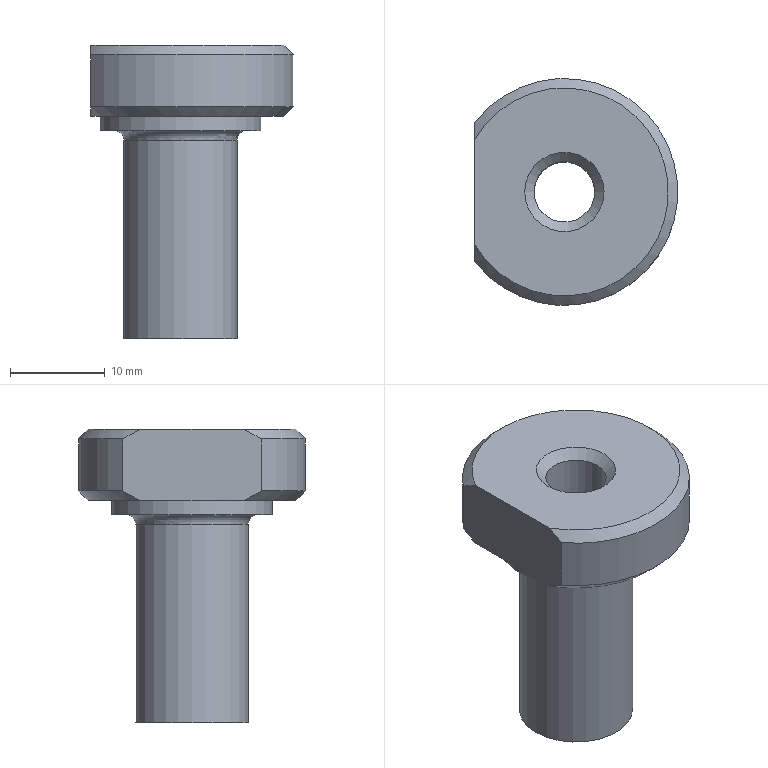Component | NX | GUIDE_BUSH_1 | 1 solid | 14 faces | box 21.5 x 24 x 31 mm | volume 4964 mm3 | plane 5 | cylinder 4 | cone 4 | torus 1 | commonest cylinder face diameters 12 x1 17 x1 24 x1 6.4 x1
STEP:
#1=CARTESIAN_POINT('',(0.,0.,0.));
#2=DIRECTION('',(0.,0.,1.));
#3=DIRECTION('',(1.,0.,0.));
#4=AXIS2_PLACEMENT_3D('',#1,#2,#3);
#5=CARTESIAN_POINT('',(-4.2,-1.,124.5));
#6=VERTEX_POINT('',#5);
#7=CARTESIAN_POINT('',(0.,-1.,124.5));
#8=DIRECTION('',(0.,0.,1.));
#9=DIRECTION('',(-1.,0.,0.));
#10=AXIS2_PLACEMENT_3D('',#7,#8,#9);
#11=CIRCLE('',#10,4.2);
#12=CARTESIAN_POINT('',(6.,-1.,124.5));
#13=DIRECTION('',(0.,0.,-1.));
#14=DIRECTION('',(-1.,0.,0.));
#15=AXIS2_PLACEMENT_3D('',#12,#13,#14);
#16=PLANE('',#15);
#17=CARTESIAN_POINT('',(10.2,0.));
#18=CARTESIAN_POINT('',(10.2,-7.275));
#19=CARTESIAN_POINT('',(3.9,-3.637));
#20=CARTESIAN_POINT('',(-2.4,-0.));
#21=CARTESIAN_POINT('',(3.9,3.637));
#22=CARTESIAN_POINT('',(10.2,7.275));
#23=CARTESIAN_POINT('',(10.2,0.));
#24=(BOUNDED_CURVE()B_SPLINE_CURVE(2,(#17,#18,#19,#20,#21,#22,#23),.UNSPECIFIED.,.T.,.F.)B_SPLINE_CURVE_WITH_KNOTS((1,2,2,2,2,1),(-2.094,0.,2.094,4.189,6.283,8.378),.UNSPECIFIED.)CURVE()GEOMETRIC_REPRESENTATION_ITEM()RATIONAL_B_SPLINE_CURVE((1.,0.5,1.,0.5,1.,0.5,1.))REPRESENTATION_ITEM(''));
#25=(GEOMETRIC_REPRESENTATION_CONTEXT(2)PARAMETRIC_REPRESENTATION_CONTEXT()REPRESENTATION_CONTEXT('',''));
#26=DEFINITIONAL_REPRESENTATION('',(#24),#25);
#27=PCURVE('',#16,#26);
#28=CARTESIAN_POINT('',(0.,-1.,124.5));
#29=DIRECTION('',(0.,0.,-1.));
#30=DIRECTION('',(-1.,0.,0.));
#31=AXIS2_PLACEMENT_3D('',#28,#29,#30);
#32=CONICAL_SURFACE('',#31,4.2,0.7854);
#33=CARTESIAN_POINT('',(6.283,0.));
#34=DIRECTION('',(-1.,0.));
#35=VECTOR('',#34,1.);
#36=LINE('',#33,#35);
#37=(GEOMETRIC_REPRESENTATION_CONTEXT(2)PARAMETRIC_REPRESENTATION_CONTEXT()REPRESENTATION_CONTEXT('',''));
#38=DEFINITIONAL_REPRESENTATION('',(#36),#37);
#39=PCURVE('',#32,#38);
#40=SURFACE_CURVE('',#11,(#27,#39),.PCURVE_S1.);
#41=EDGE_CURVE('',#6,#6,#40,.T.);
#42=ORIENTED_EDGE('',*,*,#41,.T.);
#43=EDGE_LOOP('',(#42));
#44=FACE_BOUND('',#43,.T.);
#45=CARTESIAN_POINT('',(6.,-1.,124.5));
#46=VERTEX_POINT('',#45);
#47=CARTESIAN_POINT('',(0.,-1.,124.5));
#48=DIRECTION('',(0.,0.,1.));
#49=DIRECTION('',(1.,0.,0.));
#50=AXIS2_PLACEMENT_3D('',#47,#48,#49);
#51=CIRCLE('',#50,6.);
#52=CARTESIAN_POINT('',(0.,0.));
#53=CARTESIAN_POINT('',(0.,10.392));
#54=CARTESIAN_POINT('',(9.,5.196));
#55=CARTESIAN_POINT('',(18.,0.));
#56=CARTESIAN_POINT('',(9.,-5.196));
#57=CARTESIAN_POINT('',(0.,-10.392));
#58=CARTESIAN_POINT('',(0.,0.));
#59=(BOUNDED_CURVE()B_SPLINE_CURVE(2,(#52,#53,#54,#55,#56,#57,#58),.UNSPECIFIED.,.T.,.F.)B_SPLINE_CURVE_WITH_KNOTS((1,2,2,2,2,1),(-2.094,0.,2.094,4.189,6.283,8.378),.UNSPECIFIED.)CURVE()GEOMETRIC_REPRESENTATION_ITEM()RATIONAL_B_SPLINE_CURVE((1.,0.5,1.,0.5,1.,0.5,1.))REPRESENTATION_ITEM(''));
#60=(GEOMETRIC_REPRESENTATION_CONTEXT(2)PARAMETRIC_REPRESENTATION_CONTEXT()REPRESENTATION_CONTEXT('',''));
#61=DEFINITIONAL_REPRESENTATION('',(#59),#60);
#62=PCURVE('',#16,#61);
#63=CARTESIAN_POINT('',(0.,-1.,124.5));
#64=DIRECTION('',(0.,0.,1.));
#65=DIRECTION('',(1.,0.,0.));
#66=AXIS2_PLACEMENT_3D('',#63,#64,#65);
#67=CYLINDRICAL_SURFACE('',#66,6.);
#68=CARTESIAN_POINT('',(0.,0.));
#69=DIRECTION('',(1.,0.));
#70=VECTOR('',#69,1.);
#71=LINE('',#68,#70);
#72=(GEOMETRIC_REPRESENTATION_CONTEXT(2)PARAMETRIC_REPRESENTATION_CONTEXT()REPRESENTATION_CONTEXT('',''));
#73=DEFINITIONAL_REPRESENTATION('',(#71),#72);
#74=PCURVE('',#67,#73);
#75=SURFACE_CURVE('',#51,(#62,#74),.PCURVE_S1.);
#76=EDGE_CURVE('',#46,#46,#75,.T.);
#77=ORIENTED_EDGE('',*,*,#76,.F.);
#78=EDGE_LOOP('',(#77));
#79=FACE_BOUND('',#78,.T.);
#80=ADVANCED_FACE('',(#44,#79),#16,.T.);
#81=CARTESIAN_POINT('',(-6.,-1.,145.5));
#82=VERTEX_POINT('',#81);
#83=CARTESIAN_POINT('',(6.,-1.,145.5));
#84=VERTEX_POINT('',#83);
#85=CARTESIAN_POINT('',(0.,-1.,145.5));
#86=DIRECTION('',(0.,0.,-1.));
#87=DIRECTION('',(-1.,0.,0.));
#88=AXIS2_PLACEMENT_3D('',#85,#86,#87);
#89=CIRCLE('',#88,6.);
#90=CARTESIAN_POINT('',(3.142,21.));
#91=DIRECTION('',(-1.,0.));
#92=VECTOR('',#91,1.);
#93=LINE('',#90,#92);
#94=(GEOMETRIC_REPRESENTATION_CONTEXT(2)PARAMETRIC_REPRESENTATION_CONTEXT()REPRESENTATION_CONTEXT('',''));
#95=DEFINITIONAL_REPRESENTATION('',(#93),#94);
#96=PCURVE('',#67,#95);
#97=CARTESIAN_POINT('',(0.,-1.,145.5));
#98=DIRECTION('',(0.,0.,-1.));
#99=DIRECTION('',(-1.,0.,0.));
#100=AXIS2_PLACEMENT_3D('',#97,#98,#99);
#101=TOROIDAL_SURFACE('',#100,7.,1.);
#102=CARTESIAN_POINT('',(0.,3.142));
#103=DIRECTION('',(1.,0.));
#104=VECTOR('',#103,1.);
#105=LINE('',#102,#104);
#106=(GEOMETRIC_REPRESENTATION_CONTEXT(2)PARAMETRIC_REPRESENTATION_CONTEXT()REPRESENTATION_CONTEXT('',''));
#107=DEFINITIONAL_REPRESENTATION('',(#105),#106);
#108=PCURVE('',#101,#107);
#109=SURFACE_CURVE('',#89,(#96,#108),.PCURVE_S1.);
#110=EDGE_CURVE('',#82,#84,#109,.T.);
#111=ORIENTED_EDGE('',*,*,#110,.T.);
#112=CARTESIAN_POINT('',(6.,-1.,124.5));
#113=CARTESIAN_POINT('',(6.,-1.,145.5));
#114=B_SPLINE_CURVE_WITH_KNOTS('',1,(#112,#113),.UNSPECIFIED.,.F.,.F.,(2,2),(0.,21.),.PIECEWISE_BEZIER_KNOTS.);
#115=CARTESIAN_POINT('',(0.,0.));
#116=DIRECTION('',(0.,1.));
#117=VECTOR('',#116,1.);
#118=LINE('',#115,#117);
#119=(GEOMETRIC_REPRESENTATION_CONTEXT(2)PARAMETRIC_REPRESENTATION_CONTEXT()REPRESENTATION_CONTEXT('',''));
#120=DEFINITIONAL_REPRESENTATION('',(#118),#119);
#121=PCURVE('',#67,#120);
#122=CARTESIAN_POINT('',(6.283,0.));
#123=DIRECTION('',(0.,1.));
#124=VECTOR('',#123,1.);
#125=LINE('',#122,#124);
#126=(GEOMETRIC_REPRESENTATION_CONTEXT(2)PARAMETRIC_REPRESENTATION_CONTEXT()REPRESENTATION_CONTEXT('',''));
#127=DEFINITIONAL_REPRESENTATION('',(#125),#126);
#128=PCURVE('',#67,#127);
#129=SEAM_CURVE('',#114,(#121,#128),.PCURVE_S1.);
#130=EDGE_CURVE('',#46,#84,#129,.T.);
#131=ORIENTED_EDGE('',*,*,#130,.F.);
#132=ORIENTED_EDGE('',*,*,#76,.T.);
#133=ORIENTED_EDGE('',*,*,#130,.T.);
#134=CARTESIAN_POINT('',(0.,-1.,145.5));
#135=DIRECTION('',(0.,0.,-1.));
#136=DIRECTION('',(-1.,0.,0.));
#137=AXIS2_PLACEMENT_3D('',#134,#135,#136);
#138=CIRCLE('',#137,6.);
#139=CARTESIAN_POINT('',(9.425,21.));
#140=DIRECTION('',(-1.,0.));
#141=VECTOR('',#140,1.);
#142=LINE('',#139,#141);
#143=(GEOMETRIC_REPRESENTATION_CONTEXT(2)PARAMETRIC_REPRESENTATION_CONTEXT()REPRESENTATION_CONTEXT('',''));
#144=DEFINITIONAL_REPRESENTATION('',(#142),#143);
#145=PCURVE('',#67,#144);
#146=CARTESIAN_POINT('',(0.,3.142));
#147=DIRECTION('',(1.,0.));
#148=VECTOR('',#147,1.);
#149=LINE('',#146,#148);
#150=(GEOMETRIC_REPRESENTATION_CONTEXT(2)PARAMETRIC_REPRESENTATION_CONTEXT()REPRESENTATION_CONTEXT('',''));
#151=DEFINITIONAL_REPRESENTATION('',(#149),#150);
#152=PCURVE('',#101,#151);
#153=SURFACE_CURVE('',#138,(#145,#152),.PCURVE_S1.);
#154=EDGE_CURVE('',#84,#82,#153,.T.);
#155=ORIENTED_EDGE('',*,*,#154,.T.);
#156=EDGE_LOOP('',(#111,#131,#132,#133,#155));
#157=FACE_BOUND('',#156,.T.);
#158=ADVANCED_FACE('',(#157),#67,.T.);
#159=CARTESIAN_POINT('',(-7.,-1.,146.5));
#160=VERTEX_POINT('',#159);
#161=CARTESIAN_POINT('',(0.,-1.,146.5));
#162=DIRECTION('',(0.,0.,1.));
#163=DIRECTION('',(-1.,0.,0.));
#164=AXIS2_PLACEMENT_3D('',#161,#162,#163);
#165=CIRCLE('',#164,7.);
#166=CARTESIAN_POINT('',(8.5,-1.,146.5));
#167=DIRECTION('',(0.,0.,-1.));
#168=DIRECTION('',(-1.,0.,0.));
#169=AXIS2_PLACEMENT_3D('',#166,#167,#168);
#170=PLANE('',#169);
#171=CARTESIAN_POINT('',(15.5,0.));
#172=CARTESIAN_POINT('',(15.5,-12.124));
#173=CARTESIAN_POINT('',(5.,-6.062));
#174=CARTESIAN_POINT('',(-5.5,-0.));
#175=CARTESIAN_POINT('',(5.,6.062));
#176=CARTESIAN_POINT('',(15.5,12.124));
#177=CARTESIAN_POINT('',(15.5,0.));
#178=(BOUNDED_CURVE()B_SPLINE_CURVE(2,(#171,#172,#173,#174,#175,#176,#177),.UNSPECIFIED.,.T.,.F.)B_SPLINE_CURVE_WITH_KNOTS((1,2,2,2,2,1),(-2.094,0.,2.094,4.189,6.283,8.378),.UNSPECIFIED.)CURVE()GEOMETRIC_REPRESENTATION_ITEM()RATIONAL_B_SPLINE_CURVE((1.,0.5,1.,0.5,1.,0.5,1.))REPRESENTATION_ITEM(''));
#179=(GEOMETRIC_REPRESENTATION_CONTEXT(2)PARAMETRIC_REPRESENTATION_CONTEXT()REPRESENTATION_CONTEXT('',''));
#180=DEFINITIONAL_REPRESENTATION('',(#178),#179);
#181=PCURVE('',#170,#180);
#182=CARTESIAN_POINT('',(6.283,4.712));
#183=DIRECTION('',(-1.,0.));
#184=VECTOR('',#183,1.);
#185=LINE('',#182,#184);
#186=(GEOMETRIC_REPRESENTATION_CONTEXT(2)PARAMETRIC_REPRESENTATION_CONTEXT()REPRESENTATION_CONTEXT('',''));
#187=DEFINITIONAL_REPRESENTATION('',(#185),#186);
#188=PCURVE('',#101,#187);
#189=SURFACE_CURVE('',#165,(#181,#188),.PCURVE_S1.);
#190=EDGE_CURVE('',#160,#160,#189,.T.);
#191=ORIENTED_EDGE('',*,*,#190,.T.);
#192=EDGE_LOOP('',(#191));
#193=FACE_BOUND('',#192,.T.);
#194=CARTESIAN_POINT('',(8.5,-1.,146.5));
#195=VERTEX_POINT('',#194);
#196=CARTESIAN_POINT('',(0.,-1.,146.5));
#197=DIRECTION('',(0.,0.,1.));
#198=DIRECTION('',(1.,0.,0.));
#199=AXIS2_PLACEMENT_3D('',#196,#197,#198);
#200=CIRCLE('',#199,8.5);
#201=CARTESIAN_POINT('',(0.,0.));
#202=CARTESIAN_POINT('',(0.,14.722));
#203=CARTESIAN_POINT('',(12.75,7.361));
#204=CARTESIAN_POINT('',(25.5,0.));
#205=CARTESIAN_POINT('',(12.75,-7.361));
#206=CARTESIAN_POINT('',(0.,-14.722));
#207=CARTESIAN_POINT('',(0.,0.));
#208=(BOUNDED_CURVE()B_SPLINE_CURVE(2,(#201,#202,#203,#204,#205,#206,#207),.UNSPECIFIED.,.T.,.F.)B_SPLINE_CURVE_WITH_KNOTS((1,2,2,2,2,1),(-2.094,0.,2.094,4.189,6.283,8.378),.UNSPECIFIED.)CURVE()GEOMETRIC_REPRESENTATION_ITEM()RATIONAL_B_SPLINE_CURVE((1.,0.5,1.,0.5,1.,0.5,1.))REPRESENTATION_ITEM(''));
#209=(GEOMETRIC_REPRESENTATION_CONTEXT(2)PARAMETRIC_REPRESENTATION_CONTEXT()REPRESENTATION_CONTEXT('',''));
#210=DEFINITIONAL_REPRESENTATION('',(#208),#209);
#211=PCURVE('',#170,#210);
#212=CARTESIAN_POINT('',(0.,-1.,124.5));
#213=DIRECTION('',(0.,0.,1.));
#214=DIRECTION('',(1.,0.,0.));
#215=AXIS2_PLACEMENT_3D('',#212,#213,#214);
#216=CYLINDRICAL_SURFACE('',#215,8.5);
#217=CARTESIAN_POINT('',(0.,22.));
#218=DIRECTION('',(1.,0.));
#219=VECTOR('',#218,1.);
#220=LINE('',#217,#219);
#221=(GEOMETRIC_REPRESENTATION_CONTEXT(2)PARAMETRIC_REPRESENTATION_CONTEXT()REPRESENTATION_CONTEXT('',''));
#222=DEFINITIONAL_REPRESENTATION('',(#220),#221);
#223=PCURVE('',#216,#222);
#224=SURFACE_CURVE('',#200,(#211,#223),.PCURVE_S1.);
#225=EDGE_CURVE('',#195,#195,#224,.T.);
#226=ORIENTED_EDGE('',*,*,#225,.F.);
#227=EDGE_LOOP('',(#226));
#228=FACE_BOUND('',#227,.T.);
#229=ADVANCED_FACE('',(#193,#228),#170,.T.);
#230=ORIENTED_EDGE('',*,*,#225,.T.);
#231=CARTESIAN_POINT('',(8.5,-1.,148.));
#232=VERTEX_POINT('',#231);
#233=CARTESIAN_POINT('',(8.5,-1.,146.5));
#234=CARTESIAN_POINT('',(8.5,-1.,148.));
#235=B_SPLINE_CURVE_WITH_KNOTS('',1,(#233,#234),.UNSPECIFIED.,.F.,.F.,(2,2),(22.,23.5),.PIECEWISE_BEZIER_KNOTS.);
#236=CARTESIAN_POINT('',(6.283,0.));
#237=DIRECTION('',(0.,1.));
#238=VECTOR('',#237,1.);
#239=LINE('',#236,#238);
#240=(GEOMETRIC_REPRESENTATION_CONTEXT(2)PARAMETRIC_REPRESENTATION_CONTEXT()REPRESENTATION_CONTEXT('',''));
#241=DEFINITIONAL_REPRESENTATION('',(#239),#240);
#242=PCURVE('',#216,#241);
#243=CARTESIAN_POINT('',(0.,0.));
#244=DIRECTION('',(0.,1.));
#245=VECTOR('',#244,1.);
#246=LINE('',#243,#245);
#247=(GEOMETRIC_REPRESENTATION_CONTEXT(2)PARAMETRIC_REPRESENTATION_CONTEXT()REPRESENTATION_CONTEXT('',''));
#248=DEFINITIONAL_REPRESENTATION('',(#246),#247);
#249=PCURVE('',#216,#248);
#250=SEAM_CURVE('',#235,(#242,#249),.PCURVE_S1.);
#251=EDGE_CURVE('',#195,#232,#250,.T.);
#252=ORIENTED_EDGE('',*,*,#251,.T.);
#253=CARTESIAN_POINT('',(0.,-1.,148.));
#254=DIRECTION('',(0.,0.,1.));
#255=DIRECTION('',(1.,0.,0.));
#256=AXIS2_PLACEMENT_3D('',#253,#254,#255);
#257=CIRCLE('',#256,8.5);
#258=CARTESIAN_POINT('',(0.,23.5));
#259=DIRECTION('',(1.,0.));
#260=VECTOR('',#259,1.);
#261=LINE('',#258,#260);
#262=(GEOMETRIC_REPRESENTATION_CONTEXT(2)PARAMETRIC_REPRESENTATION_CONTEXT()REPRESENTATION_CONTEXT('',''));
#263=DEFINITIONAL_REPRESENTATION('',(#261),#262);
#264=PCURVE('',#216,#263);
#265=CARTESIAN_POINT('',(12.,-1.,148.));
#266=DIRECTION('',(0.,0.,-1.));
#267=DIRECTION('',(-1.,0.,0.));
#268=AXIS2_PLACEMENT_3D('',#265,#266,#267);
#269=PLANE('',#268);
#270=CARTESIAN_POINT('',(3.5,0.));
#271=CARTESIAN_POINT('',(3.5,14.722));
#272=CARTESIAN_POINT('',(16.25,7.361));
#273=CARTESIAN_POINT('',(29.,0.));
#274=CARTESIAN_POINT('',(16.25,-7.361));
#275=CARTESIAN_POINT('',(3.5,-14.722));
#276=CARTESIAN_POINT('',(3.5,0.));
#277=(BOUNDED_CURVE()B_SPLINE_CURVE(2,(#270,#271,#272,#273,#274,#275,#276),.UNSPECIFIED.,.T.,.F.)B_SPLINE_CURVE_WITH_KNOTS((1,2,2,2,2,1),(-2.094,0.,2.094,4.189,6.283,8.378),.UNSPECIFIED.)CURVE()GEOMETRIC_REPRESENTATION_ITEM()RATIONAL_B_SPLINE_CURVE((1.,0.5,1.,0.5,1.,0.5,1.))REPRESENTATION_ITEM(''));
#278=(GEOMETRIC_REPRESENTATION_CONTEXT(2)PARAMETRIC_REPRESENTATION_CONTEXT()REPRESENTATION_CONTEXT('',''));
#279=DEFINITIONAL_REPRESENTATION('',(#277),#278);
#280=PCURVE('',#269,#279);
#281=SURFACE_CURVE('',#257,(#264,#280),.PCURVE_S1.);
#282=EDGE_CURVE('',#232,#232,#281,.T.);
#283=ORIENTED_EDGE('',*,*,#282,.F.);
#284=ORIENTED_EDGE('',*,*,#251,.F.);
#285=EDGE_LOOP('',(#230,#252,#283,#284));
#286=FACE_BOUND('',#285,.T.);
#287=ADVANCED_FACE('',(#286),#216,.T.);
#288=CARTESIAN_POINT('',(-9.5,4.545,148.));
#289=VERTEX_POINT('',#288);
#290=CARTESIAN_POINT('',(-9.5,-6.545,148.));
#291=VERTEX_POINT('',#290);
#292=CARTESIAN_POINT('',(-9.5,-1.,148.));
#293=DIRECTION('',(0.,-1.,0.));
#294=VECTOR('',#293,1.);
#295=LINE('',#292,#294);
#296=CARTESIAN_POINT('',(21.5,-0.));
#297=DIRECTION('',(-0.,-1.));
#298=VECTOR('',#297,1.);
#299=LINE('',#296,#298);
#300=(GEOMETRIC_REPRESENTATION_CONTEXT(2)PARAMETRIC_REPRESENTATION_CONTEXT()REPRESENTATION_CONTEXT('',''));
#301=DEFINITIONAL_REPRESENTATION('',(#299),#300);
#302=PCURVE('',#269,#301);
#303=CARTESIAN_POINT('',(-9.5,-8.331,124.5));
#304=DIRECTION('',(1.,0.,0.));
#305=DIRECTION('',(-0.,1.,0.));
#306=AXIS2_PLACEMENT_3D('',#303,#304,#305);
#307=PLANE('',#306);
#308=CARTESIAN_POINT('',(7.331,23.5));
#309=DIRECTION('',(-1.,0.));
#310=VECTOR('',#309,1.);
#311=LINE('',#308,#310);
#312=(GEOMETRIC_REPRESENTATION_CONTEXT(2)PARAMETRIC_REPRESENTATION_CONTEXT()REPRESENTATION_CONTEXT('',''));
#313=DEFINITIONAL_REPRESENTATION('',(#311),#312);
#314=PCURVE('',#307,#313);
#315=SURFACE_CURVE('',#295,(#302,#314),.PCURVE_S1.);
#316=EDGE_CURVE('',#289,#291,#315,.T.);
#317=ORIENTED_EDGE('',*,*,#316,.F.);
#318=CARTESIAN_POINT('',(0.,-1.,148.));
#319=DIRECTION('',(0.,0.,-1.));
#320=DIRECTION('',(-1.,0.,0.));
#321=AXIS2_PLACEMENT_3D('',#318,#319,#320);
#322=CIRCLE('',#321,11.);
#323=CARTESIAN_POINT('',(12.,0.));
#324=DIRECTION('',(1.,0.));
#325=AXIS2_PLACEMENT_2D('',#323,#324);
#326=CIRCLE('',#325,11.);
#327=(GEOMETRIC_REPRESENTATION_CONTEXT(2)PARAMETRIC_REPRESENTATION_CONTEXT()REPRESENTATION_CONTEXT('',''));
#328=DEFINITIONAL_REPRESENTATION('',(#326),#327);
#329=PCURVE('',#269,#328);
#330=CARTESIAN_POINT('',(0.,-1.,149.));
#331=DIRECTION('',(0.,0.,1.));
#332=DIRECTION('',(1.,0.,0.));
#333=AXIS2_PLACEMENT_3D('',#330,#331,#332);
#334=CONICAL_SURFACE('',#333,12.,0.7854);
#335=CARTESIAN_POINT('',(9.425,-1.));
#336=DIRECTION('',(-1.,0.));
#337=VECTOR('',#336,1.);
#338=LINE('',#335,#337);
#339=(GEOMETRIC_REPRESENTATION_CONTEXT(2)PARAMETRIC_REPRESENTATION_CONTEXT()REPRESENTATION_CONTEXT('',''));
#340=DEFINITIONAL_REPRESENTATION('',(#338),#339);
#341=PCURVE('',#334,#340);
#342=SURFACE_CURVE('',#322,(#329,#341),.PCURVE_S1.);
#343=EDGE_CURVE('',#289,#291,#342,.T.);
#344=ORIENTED_EDGE('',*,*,#343,.T.);
#345=EDGE_LOOP('',(#317,#344));
#346=FACE_BOUND('',#345,.T.);
#347=ORIENTED_EDGE('',*,*,#282,.T.);
#348=EDGE_LOOP('',(#347));
#349=FACE_BOUND('',#348,.T.);
#350=ADVANCED_FACE('',(#346,#349),#269,.T.);
#351=CARTESIAN_POINT('',(-9.5,-8.331,149.));
#352=VERTEX_POINT('',#351);
#353=CARTESIAN_POINT('',(-9.5,-8.331,154.5));
#354=VERTEX_POINT('',#353);
#355=CARTESIAN_POINT('',(-9.5,-8.331,124.5));
#356=DIRECTION('',(0.,0.,1.));
#357=VECTOR('',#356,1.);
#358=LINE('',#355,#357);
#359=CARTESIAN_POINT('',(0.,-1.,124.5));
#360=DIRECTION('',(0.,0.,1.));
#361=DIRECTION('',(1.,0.,0.));
#362=AXIS2_PLACEMENT_3D('',#359,#360,#361);
#363=CYLINDRICAL_SURFACE('',#362,12.);
#364=CARTESIAN_POINT('',(3.799,0.));
#365=DIRECTION('',(0.,1.));
#366=VECTOR('',#365,1.);
#367=LINE('',#364,#366);
#368=(GEOMETRIC_REPRESENTATION_CONTEXT(2)PARAMETRIC_REPRESENTATION_CONTEXT()REPRESENTATION_CONTEXT('',''));
#369=DEFINITIONAL_REPRESENTATION('',(#367),#368);
#370=PCURVE('',#363,#369);
#371=CARTESIAN_POINT('',(-0.,0.));
#372=DIRECTION('',(0.,1.));
#373=VECTOR('',#372,1.);
#374=LINE('',#371,#373);
#375=(GEOMETRIC_REPRESENTATION_CONTEXT(2)PARAMETRIC_REPRESENTATION_CONTEXT()REPRESENTATION_CONTEXT('',''));
#376=DEFINITIONAL_REPRESENTATION('',(#374),#375);
#377=PCURVE('',#307,#376);
#378=SURFACE_CURVE('',#358,(#370,#377),.PCURVE_S1.);
#379=EDGE_CURVE('',#352,#354,#378,.T.);
#380=ORIENTED_EDGE('',*,*,#379,.F.);
#381=CARTESIAN_POINT('',(-9.5,6.331,149.));
#382=VERTEX_POINT('',#381);
#383=CARTESIAN_POINT('',(0.,-1.,149.));
#384=DIRECTION('',(0.,0.,1.));
#385=DIRECTION('',(-1.,0.,0.));
#386=AXIS2_PLACEMENT_3D('',#383,#384,#385);
#387=CIRCLE('',#386,12.);
#388=CARTESIAN_POINT('',(3.142,24.5));
#389=DIRECTION('',(1.,0.));
#390=VECTOR('',#389,1.);
#391=LINE('',#388,#390);
#392=(GEOMETRIC_REPRESENTATION_CONTEXT(2)PARAMETRIC_REPRESENTATION_CONTEXT()REPRESENTATION_CONTEXT('',''));
#393=DEFINITIONAL_REPRESENTATION('',(#391),#392);
#394=PCURVE('',#363,#393);
#395=CARTESIAN_POINT('',(3.142,0.));
#396=DIRECTION('',(1.,0.));
#397=VECTOR('',#396,1.);
#398=LINE('',#395,#397);
#399=(GEOMETRIC_REPRESENTATION_CONTEXT(2)PARAMETRIC_REPRESENTATION_CONTEXT()REPRESENTATION_CONTEXT('',''));
#400=DEFINITIONAL_REPRESENTATION('',(#398),#399);
#401=PCURVE('',#334,#400);
#402=SURFACE_CURVE('',#387,(#394,#401),.PCURVE_S1.);
#403=EDGE_CURVE('',#352,#382,#402,.T.);
#404=ORIENTED_EDGE('',*,*,#403,.T.);
#405=CARTESIAN_POINT('',(-9.5,6.331,154.5));
#406=VERTEX_POINT('',#405);
#407=CARTESIAN_POINT('',(-9.5,6.331,124.5));
#408=DIRECTION('',(0.,0.,-1.));
#409=VECTOR('',#408,1.);
#410=LINE('',#407,#409);
#411=CARTESIAN_POINT('',(8.768,0.));
#412=DIRECTION('',(0.,-1.));
#413=VECTOR('',#412,1.);
#414=LINE('',#411,#413);
#415=(GEOMETRIC_REPRESENTATION_CONTEXT(2)PARAMETRIC_REPRESENTATION_CONTEXT()REPRESENTATION_CONTEXT('',''));
#416=DEFINITIONAL_REPRESENTATION('',(#414),#415);
#417=PCURVE('',#363,#416);
#418=CARTESIAN_POINT('',(14.663,0.));
#419=DIRECTION('',(0.,-1.));
#420=VECTOR('',#419,1.);
#421=LINE('',#418,#420);
#422=(GEOMETRIC_REPRESENTATION_CONTEXT(2)PARAMETRIC_REPRESENTATION_CONTEXT()REPRESENTATION_CONTEXT('',''));
#423=DEFINITIONAL_REPRESENTATION('',(#421),#422);
#424=PCURVE('',#307,#423);
#425=SURFACE_CURVE('',#410,(#417,#424),.PCURVE_S1.);
#426=EDGE_CURVE('',#406,#382,#425,.T.);
#427=ORIENTED_EDGE('',*,*,#426,.F.);
#428=CARTESIAN_POINT('',(0.,-1.,154.5));
#429=DIRECTION('',(0.,0.,-1.));
#430=DIRECTION('',(1.,0.,0.));
#431=AXIS2_PLACEMENT_3D('',#428,#429,#430);
#432=CIRCLE('',#431,12.);
#433=CARTESIAN_POINT('',(12.566,30.));
#434=DIRECTION('',(-1.,0.));
#435=VECTOR('',#434,1.);
#436=LINE('',#433,#435);
#437=(GEOMETRIC_REPRESENTATION_CONTEXT(2)PARAMETRIC_REPRESENTATION_CONTEXT()REPRESENTATION_CONTEXT('',''));
#438=DEFINITIONAL_REPRESENTATION('',(#436),#437);
#439=PCURVE('',#363,#438);
#440=CARTESIAN_POINT('',(0.,-1.,155.5));
#441=DIRECTION('',(0.,0.,-1.));
#442=DIRECTION('',(-1.,0.,0.));
#443=AXIS2_PLACEMENT_3D('',#440,#441,#442);
#444=CONICAL_SURFACE('',#443,11.,0.7854);
#445=CARTESIAN_POINT('',(-3.142,1.));
#446=DIRECTION('',(1.,0.));
#447=VECTOR('',#446,1.);
#448=LINE('',#445,#447);
#449=(GEOMETRIC_REPRESENTATION_CONTEXT(2)PARAMETRIC_REPRESENTATION_CONTEXT()REPRESENTATION_CONTEXT('',''));
#450=DEFINITIONAL_REPRESENTATION('',(#448),#449);
#451=PCURVE('',#444,#450);
#452=SURFACE_CURVE('',#432,(#439,#451),.PCURVE_S1.);
#453=EDGE_CURVE('',#406,#354,#452,.T.);
#454=ORIENTED_EDGE('',*,*,#453,.T.);
#455=EDGE_LOOP('',(#380,#404,#427,#454));
#456=FACE_BOUND('',#455,.T.);
#457=ADVANCED_FACE('',(#456),#363,.T.);
#458=CARTESIAN_POINT('',(-9.5,-6.545,155.5));
#459=VERTEX_POINT('',#458);
#460=CARTESIAN_POINT('',(-9.5,4.545,155.5));
#461=VERTEX_POINT('',#460);
#462=CARTESIAN_POINT('',(-9.5,-8.331,155.5));
#463=DIRECTION('',(-0.,1.,0.));
#464=VECTOR('',#463,1.);
#465=LINE('',#462,#464);
#466=CARTESIAN_POINT('',(0.,-1.,155.5));
#467=DIRECTION('',(0.,0.,1.));
#468=DIRECTION('',(1.,0.,0.));
#469=AXIS2_PLACEMENT_3D('',#466,#467,#468);
#470=PLANE('',#469);
#471=CARTESIAN_POINT('',(-9.5,-7.331));
#472=DIRECTION('',(-0.,1.));
#473=VECTOR('',#472,1.);
#474=LINE('',#471,#473);
#475=(GEOMETRIC_REPRESENTATION_CONTEXT(2)PARAMETRIC_REPRESENTATION_CONTEXT()REPRESENTATION_CONTEXT('',''));
#476=DEFINITIONAL_REPRESENTATION('',(#474),#475);
#477=PCURVE('',#470,#476);
#478=CARTESIAN_POINT('',(0.,31.));
#479=DIRECTION('',(1.,0.));
#480=VECTOR('',#479,1.);
#481=LINE('',#478,#480);
#482=(GEOMETRIC_REPRESENTATION_CONTEXT(2)PARAMETRIC_REPRESENTATION_CONTEXT()REPRESENTATION_CONTEXT('',''));
#483=DEFINITIONAL_REPRESENTATION('',(#481),#482);
#484=PCURVE('',#307,#483);
#485=SURFACE_CURVE('',#465,(#477,#484),.PCURVE_S1.);
#486=EDGE_CURVE('',#459,#461,#485,.T.);
#487=ORIENTED_EDGE('',*,*,#486,.F.);
#488=CARTESIAN_POINT('',(0.,-1.,155.5));
#489=DIRECTION('',(0.,0.,1.));
#490=DIRECTION('',(1.,0.,0.));
#491=AXIS2_PLACEMENT_3D('',#488,#489,#490);
#492=CIRCLE('',#491,11.);
#493=CARTESIAN_POINT('',(0.,0.));
#494=DIRECTION('',(1.,0.));
#495=AXIS2_PLACEMENT_2D('',#493,#494);
#496=CIRCLE('',#495,11.);
#497=(GEOMETRIC_REPRESENTATION_CONTEXT(2)PARAMETRIC_REPRESENTATION_CONTEXT()REPRESENTATION_CONTEXT('',''));
#498=DEFINITIONAL_REPRESENTATION('',(#496),#497);
#499=PCURVE('',#470,#498);
#500=CARTESIAN_POINT('',(9.425,0.));
#501=DIRECTION('',(-1.,0.));
#502=VECTOR('',#501,1.);
#503=LINE('',#500,#502);
#504=(GEOMETRIC_REPRESENTATION_CONTEXT(2)PARAMETRIC_REPRESENTATION_CONTEXT()REPRESENTATION_CONTEXT('',''));
#505=DEFINITIONAL_REPRESENTATION('',(#503),#504);
#506=PCURVE('',#444,#505);
#507=SURFACE_CURVE('',#492,(#499,#506),.PCURVE_S1.);
#508=EDGE_CURVE('',#459,#461,#507,.T.);
#509=ORIENTED_EDGE('',*,*,#508,.T.);
#510=EDGE_LOOP('',(#487,#509));
#511=FACE_BOUND('',#510,.T.);
#512=CARTESIAN_POINT('',(4.2,-1.,155.5));
#513=VERTEX_POINT('',#512);
#514=CARTESIAN_POINT('',(0.,-1.,155.5));
#515=DIRECTION('',(0.,0.,-1.));
#516=DIRECTION('',(1.,0.,0.));
#517=AXIS2_PLACEMENT_3D('',#514,#515,#516);
#518=CIRCLE('',#517,4.2);
#519=CARTESIAN_POINT('',(4.2,0.));
#520=CARTESIAN_POINT('',(4.2,-7.275));
#521=CARTESIAN_POINT('',(-2.1,-3.637));
#522=CARTESIAN_POINT('',(-8.4,-0.));
#523=CARTESIAN_POINT('',(-2.1,3.637));
#524=CARTESIAN_POINT('',(4.2,7.275));
#525=CARTESIAN_POINT('',(4.2,0.));
#526=(BOUNDED_CURVE()B_SPLINE_CURVE(2,(#519,#520,#521,#522,#523,#524,#525),.UNSPECIFIED.,.T.,.F.)B_SPLINE_CURVE_WITH_KNOTS((1,2,2,2,2,1),(-2.094,0.,2.094,4.189,6.283,8.378),.UNSPECIFIED.)CURVE()GEOMETRIC_REPRESENTATION_ITEM()RATIONAL_B_SPLINE_CURVE((1.,0.5,1.,0.5,1.,0.5,1.))REPRESENTATION_ITEM(''));
#527=(GEOMETRIC_REPRESENTATION_CONTEXT(2)PARAMETRIC_REPRESENTATION_CONTEXT()REPRESENTATION_CONTEXT('',''));
#528=DEFINITIONAL_REPRESENTATION('',(#526),#527);
#529=PCURVE('',#470,#528);
#530=CARTESIAN_POINT('',(0.,-1.,154.5));
#531=DIRECTION('',(0.,0.,1.));
#532=DIRECTION('',(1.,0.,0.));
#533=AXIS2_PLACEMENT_3D('',#530,#531,#532);
#534=CONICAL_SURFACE('',#533,3.2,0.7854);
#535=CARTESIAN_POINT('',(6.283,1.));
#536=DIRECTION('',(-1.,0.));
#537=VECTOR('',#536,1.);
#538=LINE('',#535,#537);
#539=(GEOMETRIC_REPRESENTATION_CONTEXT(2)PARAMETRIC_REPRESENTATION_CONTEXT()REPRESENTATION_CONTEXT('',''));
#540=DEFINITIONAL_REPRESENTATION('',(#538),#539);
#541=PCURVE('',#534,#540);
#542=SURFACE_CURVE('',#518,(#529,#541),.PCURVE_S1.);
#543=EDGE_CURVE('',#513,#513,#542,.T.);
#544=ORIENTED_EDGE('',*,*,#543,.T.);
#545=EDGE_LOOP('',(#544));
#546=FACE_BOUND('',#545,.T.);
#547=ADVANCED_FACE('',(#511,#546),#470,.T.);
#548=CARTESIAN_POINT('',(3.2,-1.,125.5));
#549=VERTEX_POINT('',#548);
#550=CARTESIAN_POINT('',(-3.2,-1.,125.5));
#551=VERTEX_POINT('',#550);
#552=CARTESIAN_POINT('',(0.,-1.,125.5));
#553=DIRECTION('',(0.,0.,-1.));
#554=DIRECTION('',(-1.,0.,0.));
#555=AXIS2_PLACEMENT_3D('',#552,#553,#554);
#556=CIRCLE('',#555,3.2);
#557=CARTESIAN_POINT('',(0.,-1.,124.5));
#558=DIRECTION('',(0.,0.,1.));
#559=DIRECTION('',(1.,0.,0.));
#560=AXIS2_PLACEMENT_3D('',#557,#558,#559);
#561=CYLINDRICAL_SURFACE('',#560,3.2);
#562=CARTESIAN_POINT('',(9.425,1.));
#563=DIRECTION('',(-1.,0.));
#564=VECTOR('',#563,1.);
#565=LINE('',#562,#564);
#566=(GEOMETRIC_REPRESENTATION_CONTEXT(2)PARAMETRIC_REPRESENTATION_CONTEXT()REPRESENTATION_CONTEXT('',''));
#567=DEFINITIONAL_REPRESENTATION('',(#565),#566);
#568=PCURVE('',#561,#567);
#569=CARTESIAN_POINT('',(0.,-1.));
#570=DIRECTION('',(1.,0.));
#571=VECTOR('',#570,1.);
#572=LINE('',#569,#571);
#573=(GEOMETRIC_REPRESENTATION_CONTEXT(2)PARAMETRIC_REPRESENTATION_CONTEXT()REPRESENTATION_CONTEXT('',''));
#574=DEFINITIONAL_REPRESENTATION('',(#572),#573);
#575=PCURVE('',#32,#574);
#576=SURFACE_CURVE('',#556,(#568,#575),.PCURVE_S1.);
#577=EDGE_CURVE('',#549,#551,#576,.T.);
#578=ORIENTED_EDGE('',*,*,#577,.F.);
#579=CARTESIAN_POINT('',(3.2,-1.,154.5));
#580=VERTEX_POINT('',#579);
#581=CARTESIAN_POINT('',(3.2,-1.,125.5));
#582=CARTESIAN_POINT('',(3.2,-1.,154.5));
#583=B_SPLINE_CURVE_WITH_KNOTS('',1,(#581,#582),.UNSPECIFIED.,.F.,.F.,(2,2),(1.,30.),.PIECEWISE_BEZIER_KNOTS.);
#584=CARTESIAN_POINT('',(6.283,0.));
#585=DIRECTION('',(0.,1.));
#586=VECTOR('',#585,1.);
#587=LINE('',#584,#586);
#588=(GEOMETRIC_REPRESENTATION_CONTEXT(2)PARAMETRIC_REPRESENTATION_CONTEXT()REPRESENTATION_CONTEXT('',''));
#589=DEFINITIONAL_REPRESENTATION('',(#587),#588);
#590=PCURVE('',#561,#589);
#591=CARTESIAN_POINT('',(0.,0.));
#592=DIRECTION('',(0.,1.));
#593=VECTOR('',#592,1.);
#594=LINE('',#591,#593);
#595=(GEOMETRIC_REPRESENTATION_CONTEXT(2)PARAMETRIC_REPRESENTATION_CONTEXT()REPRESENTATION_CONTEXT('',''));
#596=DEFINITIONAL_REPRESENTATION('',(#594),#595);
#597=PCURVE('',#561,#596);
#598=SEAM_CURVE('',#583,(#590,#597),.PCURVE_S1.);
#599=EDGE_CURVE('',#549,#580,#598,.T.);
#600=ORIENTED_EDGE('',*,*,#599,.T.);
#601=CARTESIAN_POINT('',(0.,-1.,154.5));
#602=DIRECTION('',(0.,0.,1.));
#603=DIRECTION('',(1.,0.,0.));
#604=AXIS2_PLACEMENT_3D('',#601,#602,#603);
#605=CIRCLE('',#604,3.2);
#606=CARTESIAN_POINT('',(0.,30.));
#607=DIRECTION('',(1.,0.));
#608=VECTOR('',#607,1.);
#609=LINE('',#606,#608);
#610=(GEOMETRIC_REPRESENTATION_CONTEXT(2)PARAMETRIC_REPRESENTATION_CONTEXT()REPRESENTATION_CONTEXT('',''));
#611=DEFINITIONAL_REPRESENTATION('',(#609),#610);
#612=PCURVE('',#561,#611);
#613=CARTESIAN_POINT('',(0.,0.));
#614=DIRECTION('',(1.,0.));
#615=VECTOR('',#614,1.);
#616=LINE('',#613,#615);
#617=(GEOMETRIC_REPRESENTATION_CONTEXT(2)PARAMETRIC_REPRESENTATION_CONTEXT()REPRESENTATION_CONTEXT('',''));
#618=DEFINITIONAL_REPRESENTATION('',(#616),#617);
#619=PCURVE('',#534,#618);
#620=SURFACE_CURVE('',#605,(#612,#619),.PCURVE_S1.);
#621=EDGE_CURVE('',#580,#580,#620,.T.);
#622=ORIENTED_EDGE('',*,*,#621,.F.);
#623=ORIENTED_EDGE('',*,*,#599,.F.);
#624=CARTESIAN_POINT('',(0.,-1.,125.5));
#625=DIRECTION('',(0.,0.,-1.));
#626=DIRECTION('',(-1.,0.,0.));
#627=AXIS2_PLACEMENT_3D('',#624,#625,#626);
#628=CIRCLE('',#627,3.2);
#629=CARTESIAN_POINT('',(3.142,1.));
#630=DIRECTION('',(-1.,0.));
#631=VECTOR('',#630,1.);
#632=LINE('',#629,#631);
#633=(GEOMETRIC_REPRESENTATION_CONTEXT(2)PARAMETRIC_REPRESENTATION_CONTEXT()REPRESENTATION_CONTEXT('',''));
#634=DEFINITIONAL_REPRESENTATION('',(#632),#633);
#635=PCURVE('',#561,#634);
#636=CARTESIAN_POINT('',(0.,-1.));
#637=DIRECTION('',(1.,0.));
#638=VECTOR('',#637,1.);
#639=LINE('',#636,#638);
#640=(GEOMETRIC_REPRESENTATION_CONTEXT(2)PARAMETRIC_REPRESENTATION_CONTEXT()REPRESENTATION_CONTEXT('',''));
#641=DEFINITIONAL_REPRESENTATION('',(#639),#640);
#642=PCURVE('',#32,#641);
#643=SURFACE_CURVE('',#628,(#635,#642),.PCURVE_S1.);
#644=EDGE_CURVE('',#551,#549,#643,.T.);
#645=ORIENTED_EDGE('',*,*,#644,.F.);
#646=EDGE_LOOP('',(#578,#600,#622,#623,#645));
#647=FACE_BOUND('',#646,.F.);
#648=ADVANCED_FACE('',(#647),#561,.F.);
#649=ORIENTED_EDGE('',*,*,#577,.T.);
#650=CARTESIAN_POINT('',(-3.2,-1.,125.5));
#651=CARTESIAN_POINT('',(-4.2,-1.,124.5));
#652=B_SPLINE_CURVE_WITH_KNOTS('',1,(#650,#651),.UNSPECIFIED.,.F.,.F.,(2,2),(-1.414,0.),.PIECEWISE_BEZIER_KNOTS.);
#653=CARTESIAN_POINT('',(6.283,0.));
#654=DIRECTION('',(0.,1.));
#655=VECTOR('',#654,1.);
#656=LINE('',#653,#655);
#657=(GEOMETRIC_REPRESENTATION_CONTEXT(2)PARAMETRIC_REPRESENTATION_CONTEXT()REPRESENTATION_CONTEXT('',''));
#658=DEFINITIONAL_REPRESENTATION('',(#656),#657);
#659=PCURVE('',#32,#658);
#660=CARTESIAN_POINT('',(0.,0.));
#661=DIRECTION('',(0.,1.));
#662=VECTOR('',#661,1.);
#663=LINE('',#660,#662);
#664=(GEOMETRIC_REPRESENTATION_CONTEXT(2)PARAMETRIC_REPRESENTATION_CONTEXT()REPRESENTATION_CONTEXT('',''));
#665=DEFINITIONAL_REPRESENTATION('',(#663),#664);
#666=PCURVE('',#32,#665);
#667=SEAM_CURVE('',#652,(#659,#666),.PCURVE_S1.);
#668=EDGE_CURVE('',#551,#6,#667,.T.);
#669=ORIENTED_EDGE('',*,*,#668,.T.);
#670=ORIENTED_EDGE('',*,*,#41,.T.);
#671=ORIENTED_EDGE('',*,*,#668,.F.);
#672=ORIENTED_EDGE('',*,*,#644,.T.);
#673=EDGE_LOOP('',(#649,#669,#670,#671,#672));
#674=FACE_BOUND('',#673,.F.);
#675=ADVANCED_FACE('',(#674),#32,.F.);
#676=ORIENTED_EDGE('',*,*,#543,.T.);
#677=CARTESIAN_POINT('',(3.2,-1.,154.5));
#678=CARTESIAN_POINT('',(4.2,-1.,155.5));
#679=B_SPLINE_CURVE_WITH_KNOTS('',1,(#677,#678),.UNSPECIFIED.,.F.,.F.,(2,2),(0.,1.414),.PIECEWISE_BEZIER_KNOTS.);
#680=CARTESIAN_POINT('',(0.,0.));
#681=DIRECTION('',(0.,1.));
#682=VECTOR('',#681,1.);
#683=LINE('',#680,#682);
#684=(GEOMETRIC_REPRESENTATION_CONTEXT(2)PARAMETRIC_REPRESENTATION_CONTEXT()REPRESENTATION_CONTEXT('',''));
#685=DEFINITIONAL_REPRESENTATION('',(#683),#684);
#686=PCURVE('',#534,#685);
#687=CARTESIAN_POINT('',(6.283,0.));
#688=DIRECTION('',(0.,1.));
#689=VECTOR('',#688,1.);
#690=LINE('',#687,#689);
#691=(GEOMETRIC_REPRESENTATION_CONTEXT(2)PARAMETRIC_REPRESENTATION_CONTEXT()REPRESENTATION_CONTEXT('',''));
#692=DEFINITIONAL_REPRESENTATION('',(#690),#691);
#693=PCURVE('',#534,#692);
#694=SEAM_CURVE('',#679,(#686,#693),.PCURVE_S1.);
#695=EDGE_CURVE('',#580,#513,#694,.T.);
#696=ORIENTED_EDGE('',*,*,#695,.F.);
#697=ORIENTED_EDGE('',*,*,#621,.T.);
#698=ORIENTED_EDGE('',*,*,#695,.T.);
#699=EDGE_LOOP('',(#676,#696,#697,#698));
#700=FACE_BOUND('',#699,.F.);
#701=ADVANCED_FACE('',(#700),#534,.F.);
#702=ORIENTED_EDGE('',*,*,#426,.T.);
#703=CARTESIAN_POINT('',(-9.5,6.331,149.));
#704=CARTESIAN_POINT('',(-9.5,5.749,148.644));
#705=CARTESIAN_POINT('',(-9.5,5.155,148.307));
#706=CARTESIAN_POINT('',(-9.5,4.545,148.));
#707=B_SPLINE_CURVE_WITH_KNOTS('',3,(#703,#704,#705,#706),.UNSPECIFIED.,.F.,.F.,(4,4),(0.,1.),.PIECEWISE_BEZIER_KNOTS.);
#708=CARTESIAN_POINT('',(14.663,24.5));
#709=CARTESIAN_POINT('',(14.081,24.144));
#710=CARTESIAN_POINT('',(13.486,23.807));
#711=CARTESIAN_POINT('',(12.877,23.5));
#712=B_SPLINE_CURVE_WITH_KNOTS('',3,(#708,#709,#710,#711),.UNSPECIFIED.,.F.,.F.,(4,4),(0.,1.),.PIECEWISE_BEZIER_KNOTS.);
#713=(GEOMETRIC_REPRESENTATION_CONTEXT(2)PARAMETRIC_REPRESENTATION_CONTEXT()REPRESENTATION_CONTEXT('',''));
#714=DEFINITIONAL_REPRESENTATION('',(#712),#713);
#715=PCURVE('',#307,#714);
#716=CARTESIAN_POINT('',(8.768,0.));
#717=CARTESIAN_POINT('',(8.896,-1.));
#718=B_SPLINE_CURVE_WITH_KNOTS('',1,(#716,#717),.UNSPECIFIED.,.F.,.F.,(2,2),(0.,1.),.PIECEWISE_BEZIER_KNOTS.);
#719=(GEOMETRIC_REPRESENTATION_CONTEXT(2)PARAMETRIC_REPRESENTATION_CONTEXT()REPRESENTATION_CONTEXT('',''));
#720=DEFINITIONAL_REPRESENTATION('',(#718),#719);
#721=PCURVE('',#334,#720);
#722=SURFACE_CURVE('',#707,(#715,#721),.PCURVE_S1.);
#723=EDGE_CURVE('',#382,#289,#722,.T.);
#724=ORIENTED_EDGE('',*,*,#723,.T.);
#725=ORIENTED_EDGE('',*,*,#316,.T.);
#726=CARTESIAN_POINT('',(-9.5,-6.545,148.));
#727=CARTESIAN_POINT('',(-9.5,-7.155,148.307));
#728=CARTESIAN_POINT('',(-9.5,-7.749,148.644));
#729=CARTESIAN_POINT('',(-9.5,-8.331,149.));
#730=B_SPLINE_CURVE_WITH_KNOTS('',3,(#726,#727,#728,#729),.UNSPECIFIED.,.F.,.F.,(4,4),(0.,1.),.PIECEWISE_BEZIER_KNOTS.);
#731=CARTESIAN_POINT('',(1.786,23.5));
#732=CARTESIAN_POINT('',(1.177,23.807));
#733=CARTESIAN_POINT('',(0.5823,24.144));
#734=CARTESIAN_POINT('',(-0.,24.5));
#735=B_SPLINE_CURVE_WITH_KNOTS('',3,(#731,#732,#733,#734),.UNSPECIFIED.,.F.,.F.,(4,4),(0.,1.),.PIECEWISE_BEZIER_KNOTS.);
#736=(GEOMETRIC_REPRESENTATION_CONTEXT(2)PARAMETRIC_REPRESENTATION_CONTEXT()REPRESENTATION_CONTEXT('',''));
#737=DEFINITIONAL_REPRESENTATION('',(#735),#736);
#738=PCURVE('',#307,#737);
#739=CARTESIAN_POINT('',(3.67,-1.));
#740=CARTESIAN_POINT('',(3.799,0.));
#741=B_SPLINE_CURVE_WITH_KNOTS('',1,(#739,#740),.UNSPECIFIED.,.F.,.F.,(2,2),(0.,1.),.PIECEWISE_BEZIER_KNOTS.);
#742=(GEOMETRIC_REPRESENTATION_CONTEXT(2)PARAMETRIC_REPRESENTATION_CONTEXT()REPRESENTATION_CONTEXT('',''));
#743=DEFINITIONAL_REPRESENTATION('',(#741),#742);
#744=PCURVE('',#334,#743);
#745=SURFACE_CURVE('',#730,(#738,#744),.PCURVE_S1.);
#746=EDGE_CURVE('',#291,#352,#745,.T.);
#747=ORIENTED_EDGE('',*,*,#746,.T.);
#748=ORIENTED_EDGE('',*,*,#379,.T.);
#749=CARTESIAN_POINT('',(-9.5,-8.331,154.5));
#750=CARTESIAN_POINT('',(-9.5,-7.749,154.856));
#751=CARTESIAN_POINT('',(-9.5,-7.155,155.193));
#752=CARTESIAN_POINT('',(-9.5,-6.545,155.5));
#753=B_SPLINE_CURVE_WITH_KNOTS('',3,(#749,#750,#751,#752),.UNSPECIFIED.,.F.,.F.,(4,4),(0.,1.),.PIECEWISE_BEZIER_KNOTS.);
#754=CARTESIAN_POINT('',(-0.,30.));
#755=CARTESIAN_POINT('',(0.5823,30.356));
#756=CARTESIAN_POINT('',(1.177,30.693));
#757=CARTESIAN_POINT('',(1.786,31.));
#758=B_SPLINE_CURVE_WITH_KNOTS('',3,(#754,#755,#756,#757),.UNSPECIFIED.,.F.,.F.,(4,4),(0.,1.),.PIECEWISE_BEZIER_KNOTS.);
#759=(GEOMETRIC_REPRESENTATION_CONTEXT(2)PARAMETRIC_REPRESENTATION_CONTEXT()REPRESENTATION_CONTEXT('',''));
#760=DEFINITIONAL_REPRESENTATION('',(#758),#759);
#761=PCURVE('',#307,#760);
#762=CARTESIAN_POINT('',(5.626,1.));
#763=CARTESIAN_POINT('',(5.755,0.));
#764=B_SPLINE_CURVE_WITH_KNOTS('',1,(#762,#763),.UNSPECIFIED.,.F.,.F.,(2,2),(0.,1.),.PIECEWISE_BEZIER_KNOTS.);
#765=(GEOMETRIC_REPRESENTATION_CONTEXT(2)PARAMETRIC_REPRESENTATION_CONTEXT()REPRESENTATION_CONTEXT('',''));
#766=DEFINITIONAL_REPRESENTATION('',(#764),#765);
#767=PCURVE('',#444,#766);
#768=SURFACE_CURVE('',#753,(#761,#767),.PCURVE_S1.);
#769=EDGE_CURVE('',#354,#459,#768,.T.);
#770=ORIENTED_EDGE('',*,*,#769,.T.);
#771=ORIENTED_EDGE('',*,*,#486,.T.);
#772=CARTESIAN_POINT('',(-9.5,4.545,155.5));
#773=CARTESIAN_POINT('',(-9.5,5.155,155.193));
#774=CARTESIAN_POINT('',(-9.5,5.749,154.856));
#775=CARTESIAN_POINT('',(-9.5,6.331,154.5));
#776=B_SPLINE_CURVE_WITH_KNOTS('',3,(#772,#773,#774,#775),.UNSPECIFIED.,.F.,.F.,(4,4),(0.,1.),.PIECEWISE_BEZIER_KNOTS.);
#777=CARTESIAN_POINT('',(12.877,31.));
#778=CARTESIAN_POINT('',(13.486,30.693));
#779=CARTESIAN_POINT('',(14.081,30.356));
#780=CARTESIAN_POINT('',(14.663,30.));
#781=B_SPLINE_CURVE_WITH_KNOTS('',3,(#777,#778,#779,#780),.UNSPECIFIED.,.F.,.F.,(4,4),(0.,1.),.PIECEWISE_BEZIER_KNOTS.);
#782=(GEOMETRIC_REPRESENTATION_CONTEXT(2)PARAMETRIC_REPRESENTATION_CONTEXT()REPRESENTATION_CONTEXT('',''));
#783=DEFINITIONAL_REPRESENTATION('',(#781),#782);
#784=PCURVE('',#307,#783);
#785=CARTESIAN_POINT('',(0.5284,0.));
#786=CARTESIAN_POINT('',(0.6573,1.));
#787=B_SPLINE_CURVE_WITH_KNOTS('',1,(#785,#786),.UNSPECIFIED.,.F.,.F.,(2,2),(0.,1.),.PIECEWISE_BEZIER_KNOTS.);
#788=(GEOMETRIC_REPRESENTATION_CONTEXT(2)PARAMETRIC_REPRESENTATION_CONTEXT()REPRESENTATION_CONTEXT('',''));
#789=DEFINITIONAL_REPRESENTATION('',(#787),#788);
#790=PCURVE('',#444,#789);
#791=SURFACE_CURVE('',#776,(#784,#790),.PCURVE_S1.);
#792=EDGE_CURVE('',#461,#406,#791,.T.);
#793=ORIENTED_EDGE('',*,*,#792,.T.);
#794=EDGE_LOOP('',(#702,#724,#725,#747,#748,#770,#771,#793));
#795=FACE_BOUND('',#794,.T.);
#796=ADVANCED_FACE('',(#795),#307,.F.);
#797=ORIENTED_EDGE('',*,*,#746,.F.);
#798=ORIENTED_EDGE('',*,*,#343,.F.);
#799=ORIENTED_EDGE('',*,*,#723,.F.);
#800=ORIENTED_EDGE('',*,*,#403,.F.);
#801=EDGE_LOOP('',(#797,#798,#799,#800));
#802=FACE_BOUND('',#801,.T.);
#803=ADVANCED_FACE('',(#802),#334,.T.);
#804=ORIENTED_EDGE('',*,*,#769,.F.);
#805=ORIENTED_EDGE('',*,*,#453,.F.);
#806=ORIENTED_EDGE('',*,*,#792,.F.);
#807=ORIENTED_EDGE('',*,*,#508,.F.);
#808=EDGE_LOOP('',(#804,#805,#806,#807));
#809=FACE_BOUND('',#808,.T.);
#810=ADVANCED_FACE('',(#809),#444,.T.);
#811=ORIENTED_EDGE('',*,*,#154,.T.);
#812=CARTESIAN_POINT('',(-6.,-1.,145.5));
#813=CARTESIAN_POINT('',(-6.,-1.,145.767));
#814=CARTESIAN_POINT('',(-6.085,-1.,146.028));
#815=CARTESIAN_POINT('',(-6.248,-1.,146.252));
#816=CARTESIAN_POINT('',(-6.472,-1.,146.415));
#817=CARTESIAN_POINT('',(-6.733,-1.,146.5));
#818=CARTESIAN_POINT('',(-7.,-1.,146.5));
#819=(BOUNDED_CURVE()B_SPLINE_CURVE(6,(#812,#813,#814,#815,#816,#817,#818),.UNSPECIFIED.,.F.,.F.)B_SPLINE_CURVE_WITH_KNOTS((7,7),(3.142,4.712),.PIECEWISE_BEZIER_KNOTS.)CURVE()GEOMETRIC_REPRESENTATION_ITEM()RATIONAL_B_SPLINE_CURVE((1.031,1.01,0.9979,0.994,0.9979,1.01,1.031))REPRESENTATION_ITEM(''));
#820=CARTESIAN_POINT('',(6.283,0.));
#821=DIRECTION('',(0.,1.));
#822=VECTOR('',#821,1.);
#823=LINE('',#820,#822);
#824=(GEOMETRIC_REPRESENTATION_CONTEXT(2)PARAMETRIC_REPRESENTATION_CONTEXT()REPRESENTATION_CONTEXT('',''));
#825=DEFINITIONAL_REPRESENTATION('',(#823),#824);
#826=PCURVE('',#101,#825);
#827=CARTESIAN_POINT('',(0.,0.));
#828=DIRECTION('',(0.,1.));
#829=VECTOR('',#828,1.);
#830=LINE('',#827,#829);
#831=(GEOMETRIC_REPRESENTATION_CONTEXT(2)PARAMETRIC_REPRESENTATION_CONTEXT()REPRESENTATION_CONTEXT('',''));
#832=DEFINITIONAL_REPRESENTATION('',(#830),#831);
#833=PCURVE('',#101,#832);
#834=SEAM_CURVE('',#819,(#826,#833),.PCURVE_S1.);
#835=EDGE_CURVE('',#82,#160,#834,.T.);
#836=ORIENTED_EDGE('',*,*,#835,.T.);
#837=ORIENTED_EDGE('',*,*,#190,.T.);
#838=ORIENTED_EDGE('',*,*,#835,.F.);
#839=ORIENTED_EDGE('',*,*,#110,.T.);
#840=EDGE_LOOP('',(#811,#836,#837,#838,#839));
#841=FACE_BOUND('',#840,.F.);
#842=ADVANCED_FACE('',(#841),#101,.F.);
#843=CLOSED_SHELL('',(#80,#158,#229,#287,#350,#457,#547,#648,#675,#701,#796,#803,#810,#842));
#844=MANIFOLD_SOLID_BREP('',#843);
#845=(LENGTH_UNIT()NAMED_UNIT(*)SI_UNIT(.MILLI.,.METRE.));
#846=UNCERTAINTY_MEASURE_WITH_UNIT(LENGTH_MEASURE(0.02),#845,'','');
#847=(NAMED_UNIT(*)PLANE_ANGLE_UNIT()SI_UNIT($,.RADIAN.));
#848=(NAMED_UNIT(*)SI_UNIT($,.STERADIAN.)SOLID_ANGLE_UNIT());
#849=(GEOMETRIC_REPRESENTATION_CONTEXT(3)GLOBAL_UNCERTAINTY_ASSIGNED_CONTEXT((#846))GLOBAL_UNIT_ASSIGNED_CONTEXT((#845,#847,#848))REPRESENTATION_CONTEXT('',''));
#850=ADVANCED_BREP_SHAPE_REPRESENTATION('',(#4,#844),#849);